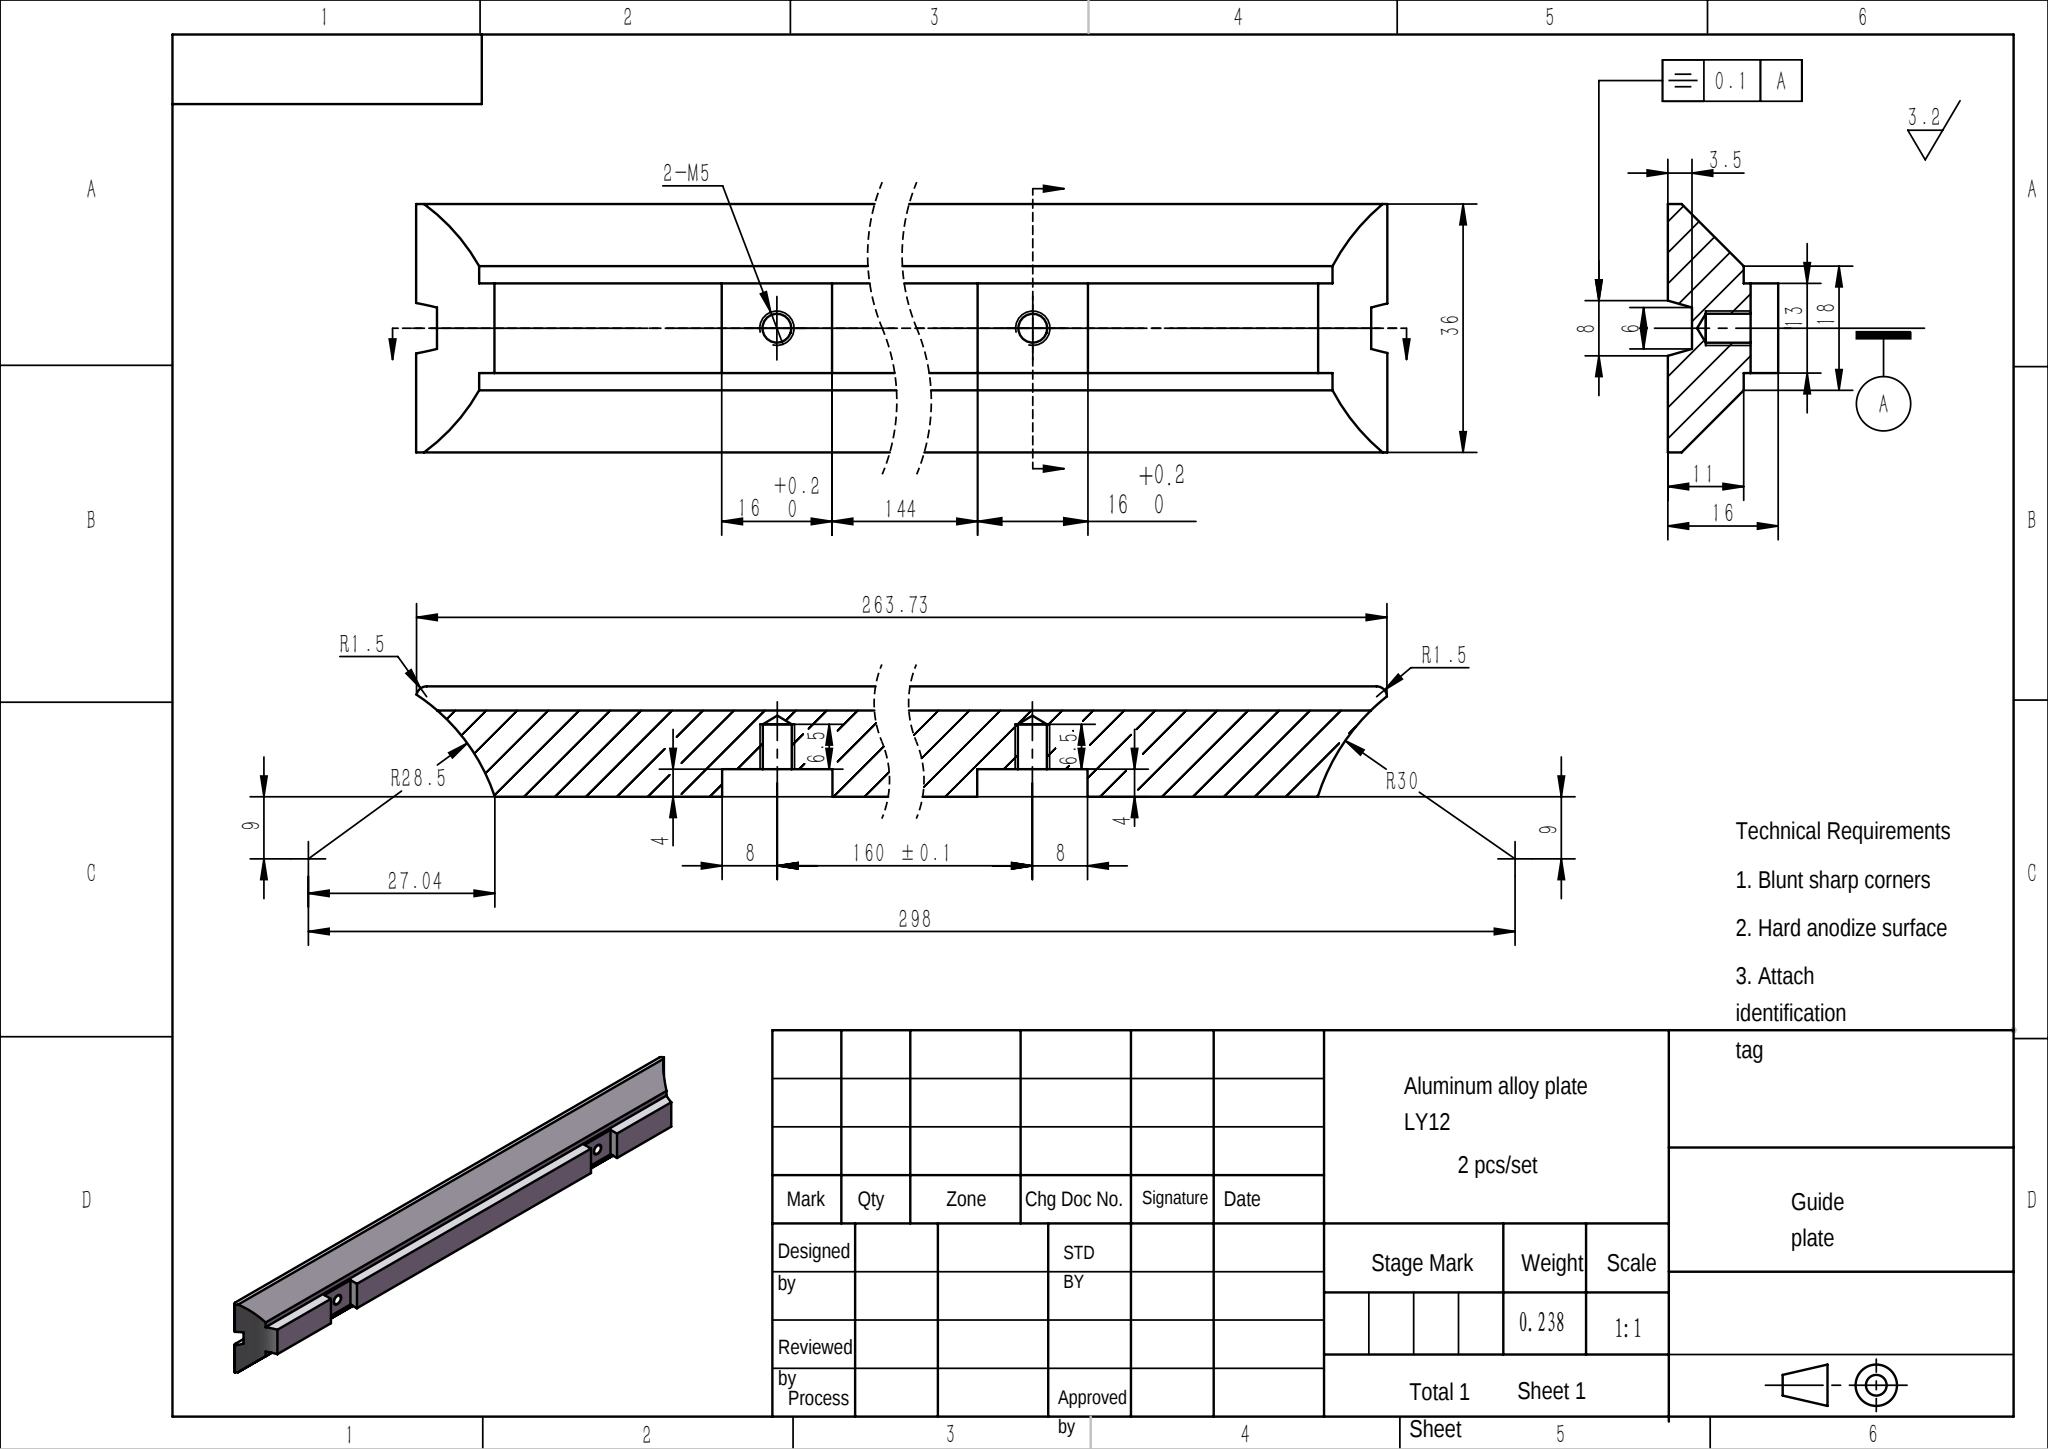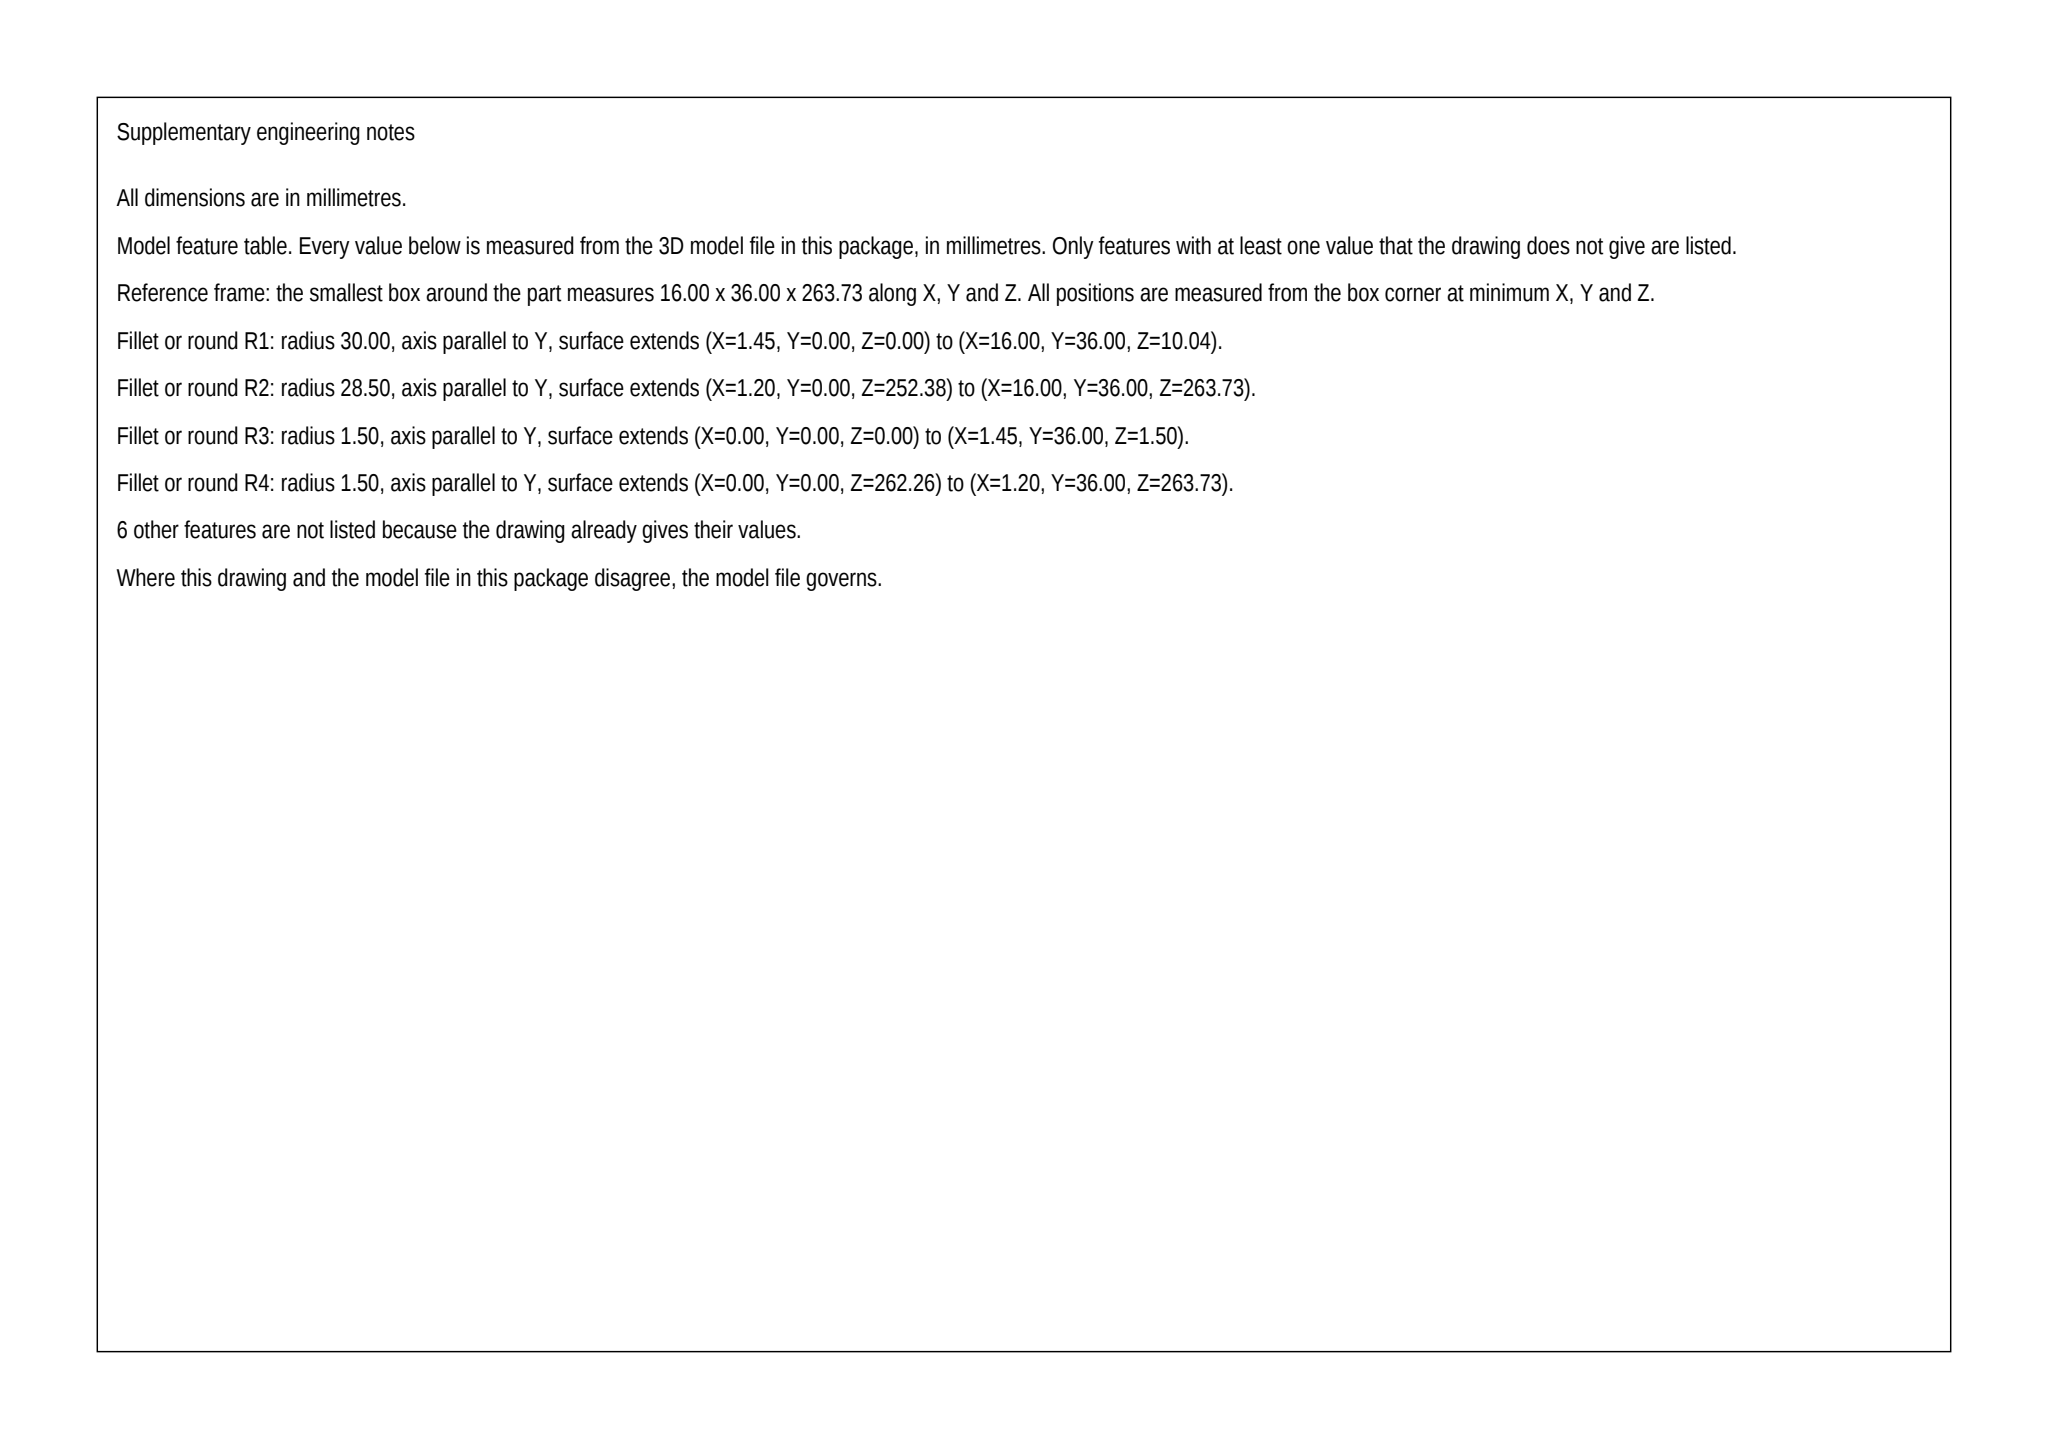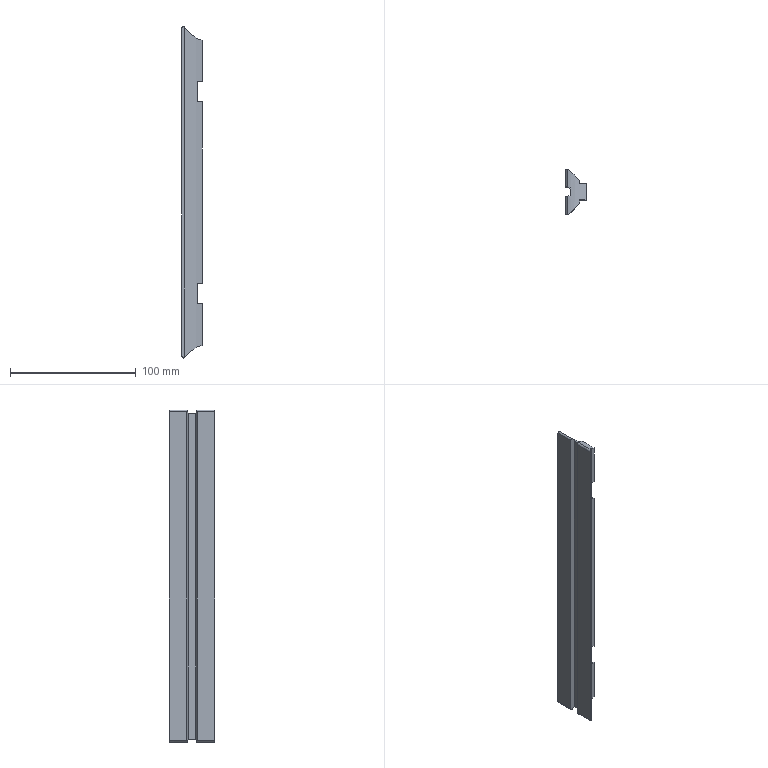Part | SolidWorks | mm | material Aluminum alloy plate LY12 | 1 solid | 36 faces | box 16 x 36 x 263.73 mm | volume 88276 mm3 | plane 22 | cylinder 10 | cone 4 | commonest cylinder face diameters 4.2 x4 3 x4 60 x1 57 x1